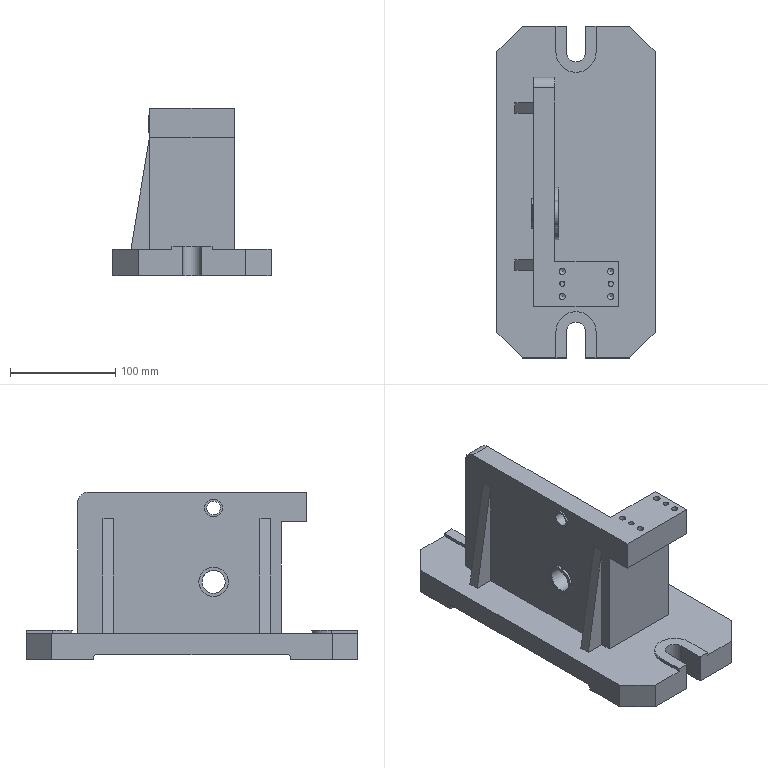Component | NX | FIXTURE_BODY | 1 solid | 98 faces | volume 1715880 mm3 | plane 46 | cylinder 26 | cone 26 | commonest cylinder face diameters 5.9 x4 3.9 x4 2.9 x4 18 x2 38 x2 6 x2 28 x2 25 x1